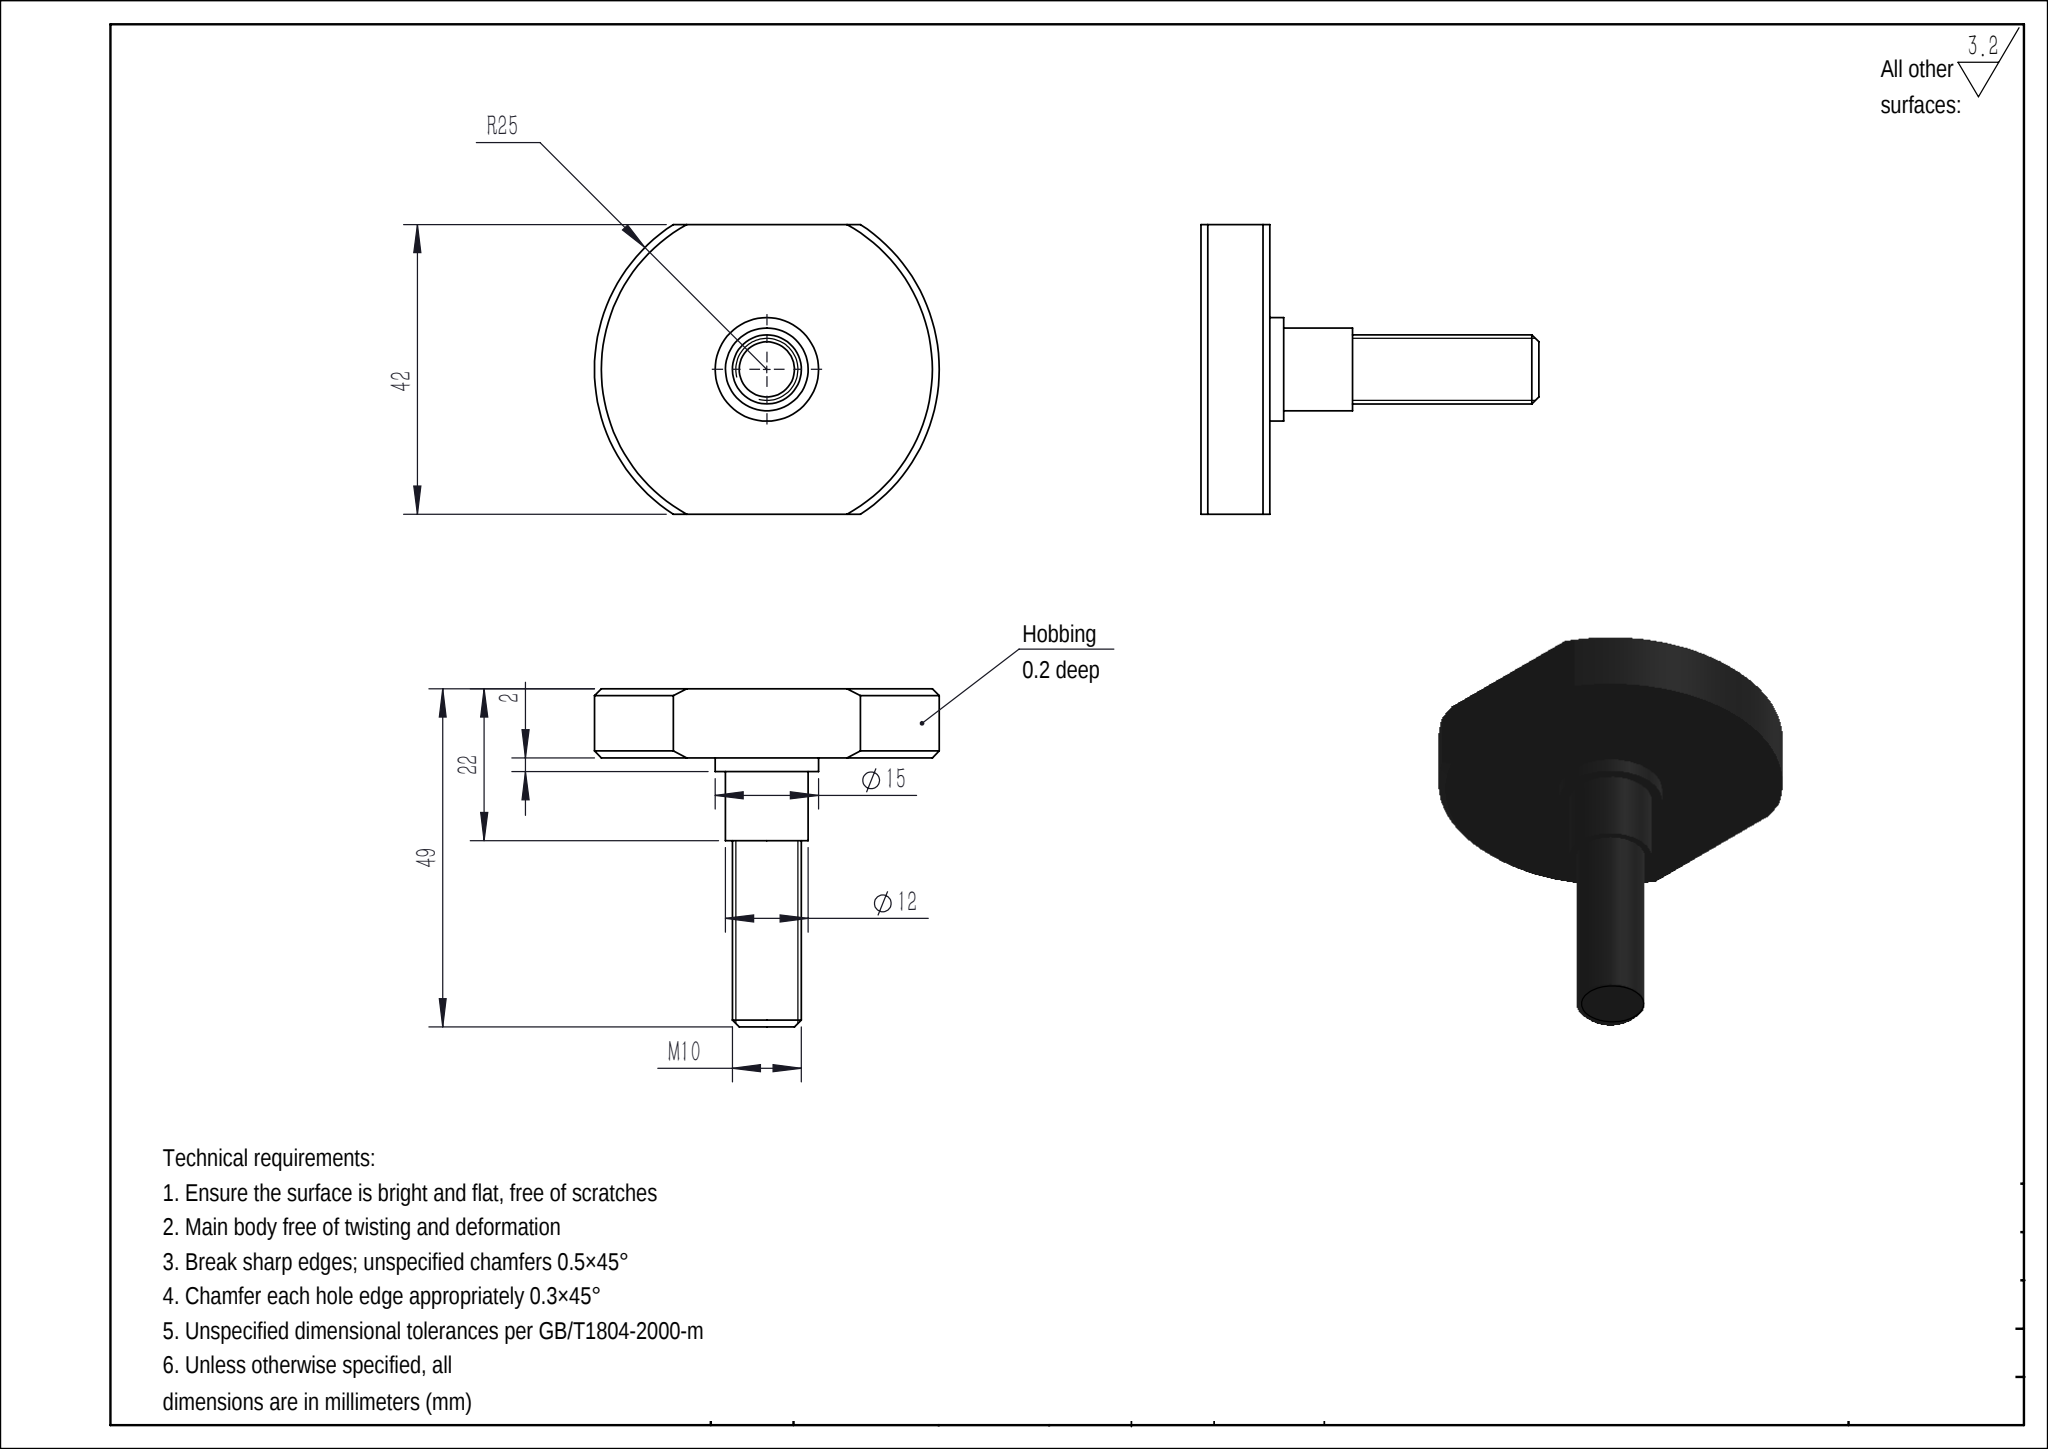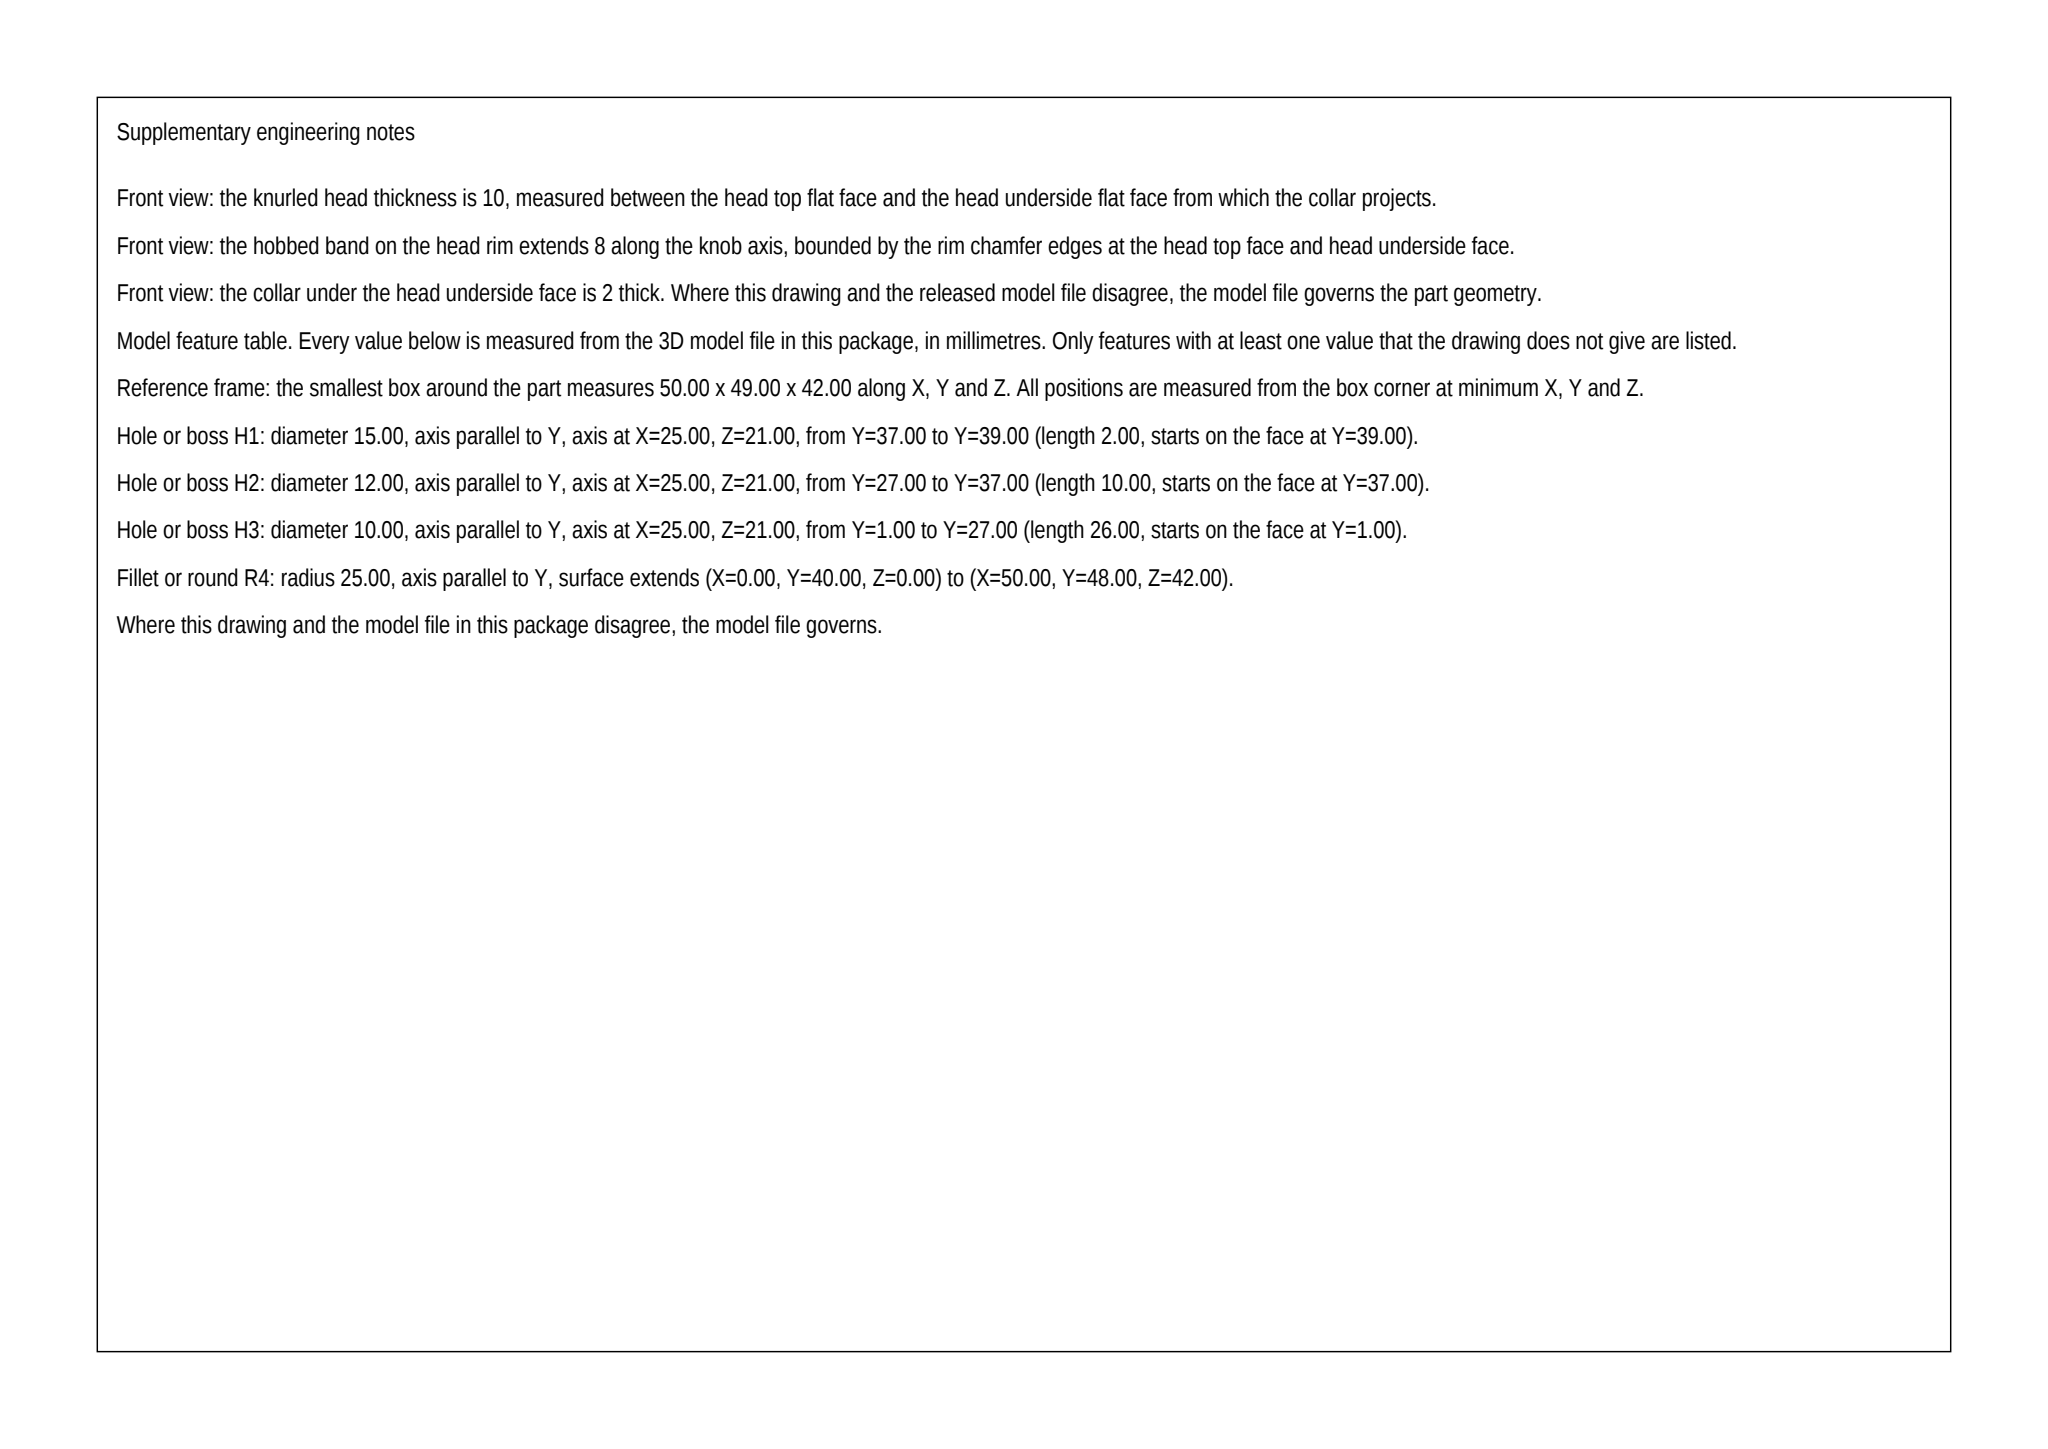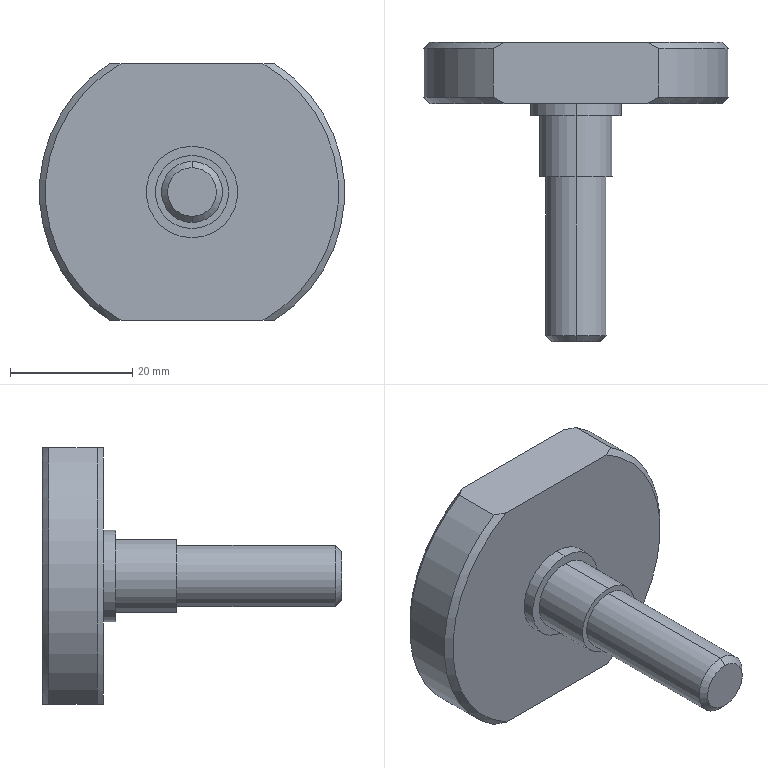Part | SolidWorks | mm | 1 solid | 21 faces | box 50 x 49 x 42 mm | volume 21653 mm3 | cylinder 8 | plane 7 | cone 6 | commonest cylinder face diameters 15 x2 12 x2 10 x2 50 x2
build123d program:
from build123d import *

# Parameters (mm, degrees)
SKETCH1_R           = 5
BOSS_EXTRUDE1_DEPTH = 27
SKETCH2_R           = 6
BOSS_EXTRUDE2_DEPTH = 12
SKETCH3_R           = 25
BOSS_EXTRUDE3_DEPTH = 10
CHAMFER1_SIZE       = 1
CHAMFER2_SIZE       = 1
SKETCH5_R           = 7.5
BOSS_EXTRUDE4_DEPTH = 2
SKETCH7_OUTSIDE_W   = 69.206
SKETCH7_OUTSIDE_H   = 69.206
SKETCH7_OUTSIDE_W_2 = 66.031
SKETCH7_OUTSIDE_H_2 = 42
CUT_EXTRUDE1_DEPTH  = 10


with BuildPart() as part:
    # Sketch1 → Boss-Extrude1 (new body)
    with BuildSketch(Plane(origin=(0, 0, 0), x_dir=(1, 0, 0), z_dir=(0, 1, 0))):
        with Locations(Location((0, 0, 0), (0, 0, 270))):
            Circle(SKETCH1_R)
    extrude(amount=BOSS_EXTRUDE1_DEPTH)

    # Sketch2 → Boss-Extrude2 (add)
    with BuildSketch(Plane(origin=(0, 27, 0), x_dir=(1, 0, 0), z_dir=(0, 1, 0))):
        with Locations(Location((0, 0, 0), (0, 0, 270))):
            Circle(SKETCH2_R)
    extrude(amount=BOSS_EXTRUDE2_DEPTH)

    # Sketch3 → Boss-Extrude3 (add)
    with BuildSketch(Plane(origin=(0, 39, 0), x_dir=(1, 0, 0), z_dir=(0, 1, 0))):
        with Locations(Location((0, 0, 0), (0, 0, 270))):
            Circle(SKETCH3_R)
    extrude(amount=BOSS_EXTRUDE3_DEPTH)

    # Chamfer1
    chamfer1_edges = [part.edges().sort_by_distance(p)[0] for p in [
        (0, 0, -5),
    ]]
    chamfer(chamfer1_edges, length=CHAMFER1_SIZE)

    # Chamfer2
    chamfer2_edges = [part.edges().sort_by_distance(p)[0] for p in [
        (0, 49, -25),
        (0, 39, -25),
    ]]
    chamfer(chamfer2_edges, length=CHAMFER2_SIZE)

    # Sketch5 → Boss-Extrude4 (add)
    with BuildSketch(Plane.XZ.offset(-39)):
        with Locations(Location((0, 0, 0), (0, 0, 90))):
            Circle(SKETCH5_R)
    extrude(amount=BOSS_EXTRUDE4_DEPTH)

    # Sketch7 outside → Cut-Extrude1 (cut)
    with BuildSketch(Plane(origin=(0, 49, 0), x_dir=(1, 0, 0), z_dir=(0, 1, 0))):
        Rectangle(SKETCH7_OUTSIDE_W, SKETCH7_OUTSIDE_H)
        Rectangle(SKETCH7_OUTSIDE_W_2, SKETCH7_OUTSIDE_H_2, mode=Mode.SUBTRACT)
    extrude(amount=-CUT_EXTRUDE1_DEPTH, mode=Mode.SUBTRACT)


solid = part.part
STEP:
#1=CARTESIAN_POINT('',(0.,37.,-7.5));
#2=VERTEX_POINT('',#1);
#3=CARTESIAN_POINT('',(0.,37.,7.5));
#4=VERTEX_POINT('',#3);
#5=CARTESIAN_POINT('',(0.,37.,0.));
#6=DIRECTION('',(0.,-1.,0.));
#7=DIRECTION('',(0.,0.,-1.));
#8=AXIS2_PLACEMENT_3D('',#5,#6,#7);
#9=CIRCLE('',#8,7.5);
#10=EDGE_CURVE('',#2,#4,#9,.T.);
#11=ORIENTED_EDGE('',*,*,#10,.F.);
#12=CARTESIAN_POINT('',(0.,39.,-7.5));
#13=VERTEX_POINT('',#12);
#14=CARTESIAN_POINT('',(0.,37.,-7.5));
#15=DIRECTION('',(0.,1.,0.));
#16=VECTOR('',#15,1000.);
#17=LINE('',#14,#16);
#18=EDGE_CURVE('',#2,#13,#17,.T.);
#19=ORIENTED_EDGE('',*,*,#18,.T.);
#20=CARTESIAN_POINT('',(0.,39.,7.5));
#21=VERTEX_POINT('',#20);
#22=CARTESIAN_POINT('',(0.,39.,0.));
#23=DIRECTION('',(0.,-1.,0.));
#24=DIRECTION('',(0.,0.,1.));
#25=AXIS2_PLACEMENT_3D('',#22,#23,#24);
#26=CIRCLE('',#25,7.5);
#27=EDGE_CURVE('',#13,#21,#26,.T.);
#28=ORIENTED_EDGE('',*,*,#27,.T.);
#29=CARTESIAN_POINT('',(0.,37.,7.5));
#30=DIRECTION('',(0.,1.,0.));
#31=VECTOR('',#30,1000.);
#32=LINE('',#29,#31);
#33=EDGE_CURVE('',#4,#21,#32,.T.);
#34=ORIENTED_EDGE('',*,*,#33,.F.);
#35=EDGE_LOOP('',(#11,#19,#28,#34));
#36=FACE_OUTER_BOUND('',#35,.T.);
#37=CARTESIAN_POINT('',(0.,37.,0.));
#38=DIRECTION('',(0.,1.,0.));
#39=DIRECTION('',(0.,0.,1.));
#40=AXIS2_PLACEMENT_3D('',#37,#38,#39);
#41=CYLINDRICAL_SURFACE('',#40,7.5);
#42=ADVANCED_FACE('',(#36),#41,.T.);
#43=CARTESIAN_POINT('',(0.,0.,-4.));
#44=VERTEX_POINT('',#43);
#45=CARTESIAN_POINT('',(0.,0.,4.));
#46=VERTEX_POINT('',#45);
#47=CARTESIAN_POINT('',(0.,0.,0.));
#48=DIRECTION('',(0.,-1.,0.));
#49=DIRECTION('',(0.,0.,1.));
#50=AXIS2_PLACEMENT_3D('',#47,#48,#49);
#51=CIRCLE('',#50,4.);
#52=EDGE_CURVE('',#44,#46,#51,.T.);
#53=ORIENTED_EDGE('',*,*,#52,.F.);
#54=CARTESIAN_POINT('',(0.,1.,-5.));
#55=VERTEX_POINT('',#54);
#56=CARTESIAN_POINT('',(0.,1.,-5.));
#57=DIRECTION('',(0.,0.7071,-0.7071));
#58=VECTOR('',#57,1000.);
#59=LINE('',#56,#58);
#60=EDGE_CURVE('',#44,#55,#59,.T.);
#61=ORIENTED_EDGE('',*,*,#60,.T.);
#62=CARTESIAN_POINT('',(0.,1.,5.));
#63=VERTEX_POINT('',#62);
#64=CARTESIAN_POINT('',(0.,1.,0.));
#65=DIRECTION('',(0.,1.,0.));
#66=DIRECTION('',(0.,0.,1.));
#67=AXIS2_PLACEMENT_3D('',#64,#65,#66);
#68=CIRCLE('',#67,5.);
#69=EDGE_CURVE('',#63,#55,#68,.T.);
#70=ORIENTED_EDGE('',*,*,#69,.F.);
#71=CARTESIAN_POINT('',(0.,1.,5.));
#72=DIRECTION('',(0.,0.7071,0.7071));
#73=VECTOR('',#72,1000.);
#74=LINE('',#71,#73);
#75=EDGE_CURVE('',#46,#63,#74,.T.);
#76=ORIENTED_EDGE('',*,*,#75,.F.);
#77=EDGE_LOOP('',(#53,#61,#70,#76));
#78=FACE_OUTER_BOUND('',#77,.T.);
#79=CARTESIAN_POINT('',(0.,1.,0.));
#80=DIRECTION('',(0.,1.,0.));
#81=DIRECTION('',(0.,0.,1.));
#82=AXIS2_PLACEMENT_3D('',#79,#80,#81);
#83=CONICAL_SURFACE('',#82,5.,0.7854);
#84=ADVANCED_FACE('',(#78),#83,.T.);
#85=CARTESIAN_POINT('',(0.,37.,-6.));
#86=VERTEX_POINT('',#85);
#87=CARTESIAN_POINT('',(0.,37.,6.));
#88=VERTEX_POINT('',#87);
#89=CARTESIAN_POINT('',(0.,37.,0.));
#90=DIRECTION('',(0.,-1.,0.));
#91=DIRECTION('',(0.,0.,-1.));
#92=AXIS2_PLACEMENT_3D('',#89,#90,#91);
#93=CIRCLE('',#92,6.);
#94=EDGE_CURVE('',#86,#88,#93,.T.);
#95=ORIENTED_EDGE('',*,*,#94,.T.);
#96=CARTESIAN_POINT('',(0.,27.,6.));
#97=VERTEX_POINT('',#96);
#98=CARTESIAN_POINT('',(0.,39.,6.));
#99=DIRECTION('',(0.,-1.,0.));
#100=VECTOR('',#99,1000.);
#101=LINE('',#98,#100);
#102=EDGE_CURVE('',#88,#97,#101,.T.);
#103=ORIENTED_EDGE('',*,*,#102,.T.);
#104=CARTESIAN_POINT('',(0.,27.,-6.));
#105=VERTEX_POINT('',#104);
#106=CARTESIAN_POINT('',(0.,27.,0.));
#107=DIRECTION('',(0.,1.,0.));
#108=DIRECTION('',(0.,0.,1.));
#109=AXIS2_PLACEMENT_3D('',#106,#107,#108);
#110=CIRCLE('',#109,6.);
#111=EDGE_CURVE('',#97,#105,#110,.T.);
#112=ORIENTED_EDGE('',*,*,#111,.T.);
#113=CARTESIAN_POINT('',(0.,39.,-6.));
#114=DIRECTION('',(0.,-1.,0.));
#115=VECTOR('',#114,1000.);
#116=LINE('',#113,#115);
#117=EDGE_CURVE('',#86,#105,#116,.T.);
#118=ORIENTED_EDGE('',*,*,#117,.F.);
#119=EDGE_LOOP('',(#95,#103,#112,#118));
#120=FACE_OUTER_BOUND('',#119,.T.);
#121=CARTESIAN_POINT('',(0.,39.,0.));
#122=DIRECTION('',(0.,-1.,0.));
#123=DIRECTION('',(0.,0.,-1.));
#124=AXIS2_PLACEMENT_3D('',#121,#122,#123);
#125=CYLINDRICAL_SURFACE('',#124,6.);
#126=ADVANCED_FACE('',(#120),#125,.T.);
#127=CARTESIAN_POINT('',(0.,27.,5.));
#128=VERTEX_POINT('',#127);
#129=CARTESIAN_POINT('',(0.,27.,-5.));
#130=VERTEX_POINT('',#129);
#131=CARTESIAN_POINT('',(0.,27.,0.));
#132=DIRECTION('',(0.,1.,0.));
#133=DIRECTION('',(0.,0.,1.));
#134=AXIS2_PLACEMENT_3D('',#131,#132,#133);
#135=CIRCLE('',#134,5.);
#136=EDGE_CURVE('',#128,#130,#135,.T.);
#137=ORIENTED_EDGE('',*,*,#136,.F.);
#138=CARTESIAN_POINT('',(0.,27.,5.));
#139=DIRECTION('',(0.,-1.,0.));
#140=VECTOR('',#139,1000.);
#141=LINE('',#138,#140);
#142=EDGE_CURVE('',#128,#63,#141,.T.);
#143=ORIENTED_EDGE('',*,*,#142,.T.);
#144=ORIENTED_EDGE('',*,*,#69,.T.);
#145=CARTESIAN_POINT('',(0.,27.,-5.));
#146=DIRECTION('',(0.,-1.,0.));
#147=VECTOR('',#146,1000.);
#148=LINE('',#145,#147);
#149=EDGE_CURVE('',#130,#55,#148,.T.);
#150=ORIENTED_EDGE('',*,*,#149,.F.);
#151=EDGE_LOOP('',(#137,#143,#144,#150));
#152=FACE_OUTER_BOUND('',#151,.T.);
#153=CARTESIAN_POINT('',(0.,27.,0.));
#154=DIRECTION('',(0.,-1.,0.));
#155=DIRECTION('',(0.,0.,-1.));
#156=AXIS2_PLACEMENT_3D('',#153,#154,#155);
#157=CYLINDRICAL_SURFACE('',#156,5.);
#158=ADVANCED_FACE('',(#152),#157,.T.);
#159=CARTESIAN_POINT('',(-11.619,49.,-21.));
#160=VERTEX_POINT('',#159);
#161=CARTESIAN_POINT('',(-11.619,49.,21.));
#162=VERTEX_POINT('',#161);
#163=CARTESIAN_POINT('',(0.,49.,0.));
#164=DIRECTION('',(0.,1.,0.));
#165=DIRECTION('',(0.,0.,1.));
#166=AXIS2_PLACEMENT_3D('',#163,#164,#165);
#167=CIRCLE('',#166,24.);
#168=EDGE_CURVE('',#160,#162,#167,.T.);
#169=ORIENTED_EDGE('',*,*,#168,.T.);
#170=CARTESIAN_POINT('',(11.619,49.,21.));
#171=VERTEX_POINT('',#170);
#172=CARTESIAN_POINT('',(-33.015,49.,21.));
#173=DIRECTION('',(1.,0.,0.));
#174=VECTOR('',#173,1000.);
#175=LINE('',#172,#174);
#176=EDGE_CURVE('',#162,#171,#175,.T.);
#177=ORIENTED_EDGE('',*,*,#176,.T.);
#178=CARTESIAN_POINT('',(11.619,49.,-21.));
#179=VERTEX_POINT('',#178);
#180=CARTESIAN_POINT('',(0.,49.,0.));
#181=DIRECTION('',(0.,1.,0.));
#182=DIRECTION('',(0.,0.,1.));
#183=AXIS2_PLACEMENT_3D('',#180,#181,#182);
#184=CIRCLE('',#183,24.);
#185=EDGE_CURVE('',#171,#179,#184,.T.);
#186=ORIENTED_EDGE('',*,*,#185,.T.);
#187=CARTESIAN_POINT('',(-33.015,49.,-21.));
#188=DIRECTION('',(-1.,0.,0.));
#189=VECTOR('',#188,1000.);
#190=LINE('',#187,#189);
#191=EDGE_CURVE('',#179,#160,#190,.T.);
#192=ORIENTED_EDGE('',*,*,#191,.T.);
#193=EDGE_LOOP('',(#169,#177,#186,#192));
#194=FACE_OUTER_BOUND('',#193,.T.);
#195=CARTESIAN_POINT('',(0.,49.,0.));
#196=DIRECTION('',(0.,1.,0.));
#197=DIRECTION('',(0.,0.,1.));
#198=AXIS2_PLACEMENT_3D('',#195,#196,#197);
#199=PLANE('',#198);
#200=ADVANCED_FACE('',(#194),#199,.T.);
#201=CARTESIAN_POINT('',(-13.565,48.,21.));
#202=VERTEX_POINT('',#201);
#203=CARTESIAN_POINT('',(-13.565,48.,-21.));
#204=VERTEX_POINT('',#203);
#205=CARTESIAN_POINT('',(0.,48.,0.));
#206=DIRECTION('',(0.,-1.,0.));
#207=DIRECTION('',(0.,0.,1.));
#208=AXIS2_PLACEMENT_3D('',#205,#206,#207);
#209=CIRCLE('',#208,25.);
#210=EDGE_CURVE('',#202,#204,#209,.T.);
#211=ORIENTED_EDGE('',*,*,#210,.F.);
#212=CARTESIAN_POINT('',(-13.565,48.,21.));
#213=CARTESIAN_POINT('',(-12.923,48.348,21.));
#214=CARTESIAN_POINT('',(-12.275,48.682,21.));
#215=CARTESIAN_POINT('',(-11.619,49.,21.));
#216=B_SPLINE_CURVE_WITH_KNOTS('',3,(#212,#213,#214,#215),.UNSPECIFIED.,.F.,.F.,(4,4),(0.04795,0.05014),.UNSPECIFIED.);
#217=EDGE_CURVE('',#202,#162,#216,.T.);
#218=ORIENTED_EDGE('',*,*,#217,.T.);
#219=ORIENTED_EDGE('',*,*,#168,.F.);
#220=CARTESIAN_POINT('',(-11.619,49.,-21.));
#221=CARTESIAN_POINT('',(-12.276,48.682,-21.));
#222=CARTESIAN_POINT('',(-12.924,48.347,-21.));
#223=CARTESIAN_POINT('',(-13.565,48.,-21.));
#224=B_SPLINE_CURVE_WITH_KNOTS('',3,(#220,#221,#222,#223),.UNSPECIFIED.,.F.,.F.,(4,4),(0.07437,0.07658),.UNSPECIFIED.);
#225=EDGE_CURVE('',#160,#204,#224,.T.);
#226=ORIENTED_EDGE('',*,*,#225,.T.);
#227=EDGE_LOOP('',(#211,#218,#219,#226));
#228=FACE_OUTER_BOUND('',#227,.T.);
#229=CARTESIAN_POINT('',(0.,49.,0.));
#230=DIRECTION('',(0.,-1.,0.));
#231=DIRECTION('',(0.,0.,-1.));
#232=AXIS2_PLACEMENT_3D('',#229,#230,#231);
#233=CONICAL_SURFACE('',#232,24.,0.7854);
#234=ADVANCED_FACE('',(#228),#233,.T.);
#235=ORIENTED_EDGE('',*,*,#185,.F.);
#236=CARTESIAN_POINT('',(13.565,48.,21.));
#237=VERTEX_POINT('',#236);
#238=CARTESIAN_POINT('',(11.619,49.,21.));
#239=CARTESIAN_POINT('',(12.276,48.682,21.));
#240=CARTESIAN_POINT('',(12.924,48.347,21.));
#241=CARTESIAN_POINT('',(13.565,48.,21.));
#242=B_SPLINE_CURVE_WITH_KNOTS('',3,(#238,#239,#240,#241),.UNSPECIFIED.,.F.,.F.,(4,4),(0.07437,0.07658),.UNSPECIFIED.);
#243=EDGE_CURVE('',#171,#237,#242,.T.);
#244=ORIENTED_EDGE('',*,*,#243,.T.);
#245=CARTESIAN_POINT('',(13.565,48.,-21.));
#246=VERTEX_POINT('',#245);
#247=CARTESIAN_POINT('',(0.,48.,0.));
#248=DIRECTION('',(0.,-1.,0.));
#249=DIRECTION('',(0.,0.,1.));
#250=AXIS2_PLACEMENT_3D('',#247,#248,#249);
#251=CIRCLE('',#250,25.);
#252=EDGE_CURVE('',#246,#237,#251,.T.);
#253=ORIENTED_EDGE('',*,*,#252,.F.);
#254=CARTESIAN_POINT('',(13.565,48.,-21.));
#255=CARTESIAN_POINT('',(12.923,48.348,-21.));
#256=CARTESIAN_POINT('',(12.275,48.682,-21.));
#257=CARTESIAN_POINT('',(11.619,49.,-21.));
#258=B_SPLINE_CURVE_WITH_KNOTS('',3,(#254,#255,#256,#257),.UNSPECIFIED.,.F.,.F.,(4,4),(0.04795,0.05014),.UNSPECIFIED.);
#259=EDGE_CURVE('',#246,#179,#258,.T.);
#260=ORIENTED_EDGE('',*,*,#259,.T.);
#261=EDGE_LOOP('',(#235,#244,#253,#260));
#262=FACE_OUTER_BOUND('',#261,.T.);
#263=CARTESIAN_POINT('',(0.,49.,0.));
#264=DIRECTION('',(0.,-1.,0.));
#265=DIRECTION('',(0.,0.,-1.));
#266=AXIS2_PLACEMENT_3D('',#263,#264,#265);
#267=CONICAL_SURFACE('',#266,24.,0.7854);
#268=ADVANCED_FACE('',(#262),#267,.T.);
#269=CARTESIAN_POINT('',(-13.565,40.,21.));
#270=VERTEX_POINT('',#269);
#271=CARTESIAN_POINT('',(-13.565,49.,21.));
#272=DIRECTION('',(0.,-1.,0.));
#273=VECTOR('',#272,1000.);
#274=LINE('',#271,#273);
#275=EDGE_CURVE('',#202,#270,#274,.T.);
#276=ORIENTED_EDGE('',*,*,#275,.F.);
#277=ORIENTED_EDGE('',*,*,#210,.T.);
#278=CARTESIAN_POINT('',(-13.565,40.,-21.));
#279=VERTEX_POINT('',#278);
#280=CARTESIAN_POINT('',(-13.565,49.,-21.));
#281=DIRECTION('',(0.,1.,0.));
#282=VECTOR('',#281,1000.);
#283=LINE('',#280,#282);
#284=EDGE_CURVE('',#279,#204,#283,.T.);
#285=ORIENTED_EDGE('',*,*,#284,.F.);
#286=CARTESIAN_POINT('',(0.,40.,0.));
#287=DIRECTION('',(0.,1.,0.));
#288=DIRECTION('',(0.,0.,1.));
#289=AXIS2_PLACEMENT_3D('',#286,#287,#288);
#290=CIRCLE('',#289,25.);
#291=EDGE_CURVE('',#279,#270,#290,.T.);
#292=ORIENTED_EDGE('',*,*,#291,.T.);
#293=EDGE_LOOP('',(#276,#277,#285,#292));
#294=FACE_OUTER_BOUND('',#293,.T.);
#295=CARTESIAN_POINT('',(0.,49.,0.));
#296=DIRECTION('',(0.,-1.,0.));
#297=DIRECTION('',(0.,0.,-1.));
#298=AXIS2_PLACEMENT_3D('',#295,#296,#297);
#299=CYLINDRICAL_SURFACE('',#298,25.);
#300=ADVANCED_FACE('',(#294),#299,.T.);
#301=CARTESIAN_POINT('',(13.565,40.,21.));
#302=VERTEX_POINT('',#301);
#303=CARTESIAN_POINT('',(13.565,49.,21.));
#304=DIRECTION('',(0.,1.,0.));
#305=VECTOR('',#304,1000.);
#306=LINE('',#303,#305);
#307=EDGE_CURVE('',#302,#237,#306,.T.);
#308=ORIENTED_EDGE('',*,*,#307,.F.);
#309=CARTESIAN_POINT('',(13.565,40.,-21.));
#310=VERTEX_POINT('',#309);
#311=CARTESIAN_POINT('',(0.,40.,0.));
#312=DIRECTION('',(0.,1.,0.));
#313=DIRECTION('',(0.,0.,1.));
#314=AXIS2_PLACEMENT_3D('',#311,#312,#313);
#315=CIRCLE('',#314,25.);
#316=EDGE_CURVE('',#302,#310,#315,.T.);
#317=ORIENTED_EDGE('',*,*,#316,.T.);
#318=CARTESIAN_POINT('',(13.565,49.,-21.));
#319=DIRECTION('',(0.,-1.,0.));
#320=VECTOR('',#319,1000.);
#321=LINE('',#318,#320);
#322=EDGE_CURVE('',#246,#310,#321,.T.);
#323=ORIENTED_EDGE('',*,*,#322,.F.);
#324=ORIENTED_EDGE('',*,*,#252,.T.);
#325=EDGE_LOOP('',(#308,#317,#323,#324));
#326=FACE_OUTER_BOUND('',#325,.T.);
#327=CARTESIAN_POINT('',(0.,49.,0.));
#328=DIRECTION('',(0.,-1.,0.));
#329=DIRECTION('',(0.,0.,-1.));
#330=AXIS2_PLACEMENT_3D('',#327,#328,#329);
#331=CYLINDRICAL_SURFACE('',#330,25.);
#332=ADVANCED_FACE('',(#326),#331,.T.);
#333=ORIENTED_EDGE('',*,*,#316,.F.);
#334=CARTESIAN_POINT('',(11.619,39.,21.));
#335=VERTEX_POINT('',#334);
#336=CARTESIAN_POINT('',(13.565,40.,21.));
#337=CARTESIAN_POINT('',(12.923,39.652,21.));
#338=CARTESIAN_POINT('',(12.275,39.318,21.));
#339=CARTESIAN_POINT('',(11.619,39.,21.));
#340=B_SPLINE_CURVE_WITH_KNOTS('',3,(#336,#337,#338,#339),.UNSPECIFIED.,.F.,.F.,(4,4),(0.04795,0.05014),.UNSPECIFIED.);
#341=EDGE_CURVE('',#302,#335,#340,.T.);
#342=ORIENTED_EDGE('',*,*,#341,.T.);
#343=CARTESIAN_POINT('',(11.619,39.,-21.));
#344=VERTEX_POINT('',#343);
#345=CARTESIAN_POINT('',(0.,39.,0.));
#346=DIRECTION('',(0.,-1.,0.));
#347=DIRECTION('',(0.,0.,1.));
#348=AXIS2_PLACEMENT_3D('',#345,#346,#347);
#349=CIRCLE('',#348,24.);
#350=EDGE_CURVE('',#344,#335,#349,.T.);
#351=ORIENTED_EDGE('',*,*,#350,.F.);
#352=CARTESIAN_POINT('',(11.619,39.,-21.));
#353=CARTESIAN_POINT('',(12.276,39.318,-21.));
#354=CARTESIAN_POINT('',(12.924,39.653,-21.));
#355=CARTESIAN_POINT('',(13.565,40.,-21.));
#356=B_SPLINE_CURVE_WITH_KNOTS('',3,(#352,#353,#354,#355),.UNSPECIFIED.,.F.,.F.,(4,4),(0.07437,0.07658),.UNSPECIFIED.);
#357=EDGE_CURVE('',#344,#310,#356,.T.);
#358=ORIENTED_EDGE('',*,*,#357,.T.);
#359=EDGE_LOOP('',(#333,#342,#351,#358));
#360=FACE_OUTER_BOUND('',#359,.T.);
#361=CARTESIAN_POINT('',(0.,40.,0.));
#362=DIRECTION('',(0.,1.,0.));
#363=DIRECTION('',(0.,0.,1.));
#364=AXIS2_PLACEMENT_3D('',#361,#362,#363);
#365=CONICAL_SURFACE('',#364,25.,0.7854);
#366=ADVANCED_FACE('',(#360),#365,.T.);
#367=CARTESIAN_POINT('',(-11.619,39.,21.));
#368=VERTEX_POINT('',#367);
#369=CARTESIAN_POINT('',(-11.619,39.,-21.));
#370=VERTEX_POINT('',#369);
#371=CARTESIAN_POINT('',(0.,39.,0.));
#372=DIRECTION('',(0.,-1.,0.));
#373=DIRECTION('',(0.,0.,1.));
#374=AXIS2_PLACEMENT_3D('',#371,#372,#373);
#375=CIRCLE('',#374,24.);
#376=EDGE_CURVE('',#368,#370,#375,.T.);
#377=ORIENTED_EDGE('',*,*,#376,.F.);
#378=CARTESIAN_POINT('',(-11.619,39.,21.));
#379=CARTESIAN_POINT('',(-12.276,39.318,21.));
#380=CARTESIAN_POINT('',(-12.924,39.653,21.));
#381=CARTESIAN_POINT('',(-13.565,40.,21.));
#382=B_SPLINE_CURVE_WITH_KNOTS('',3,(#378,#379,#380,#381),.UNSPECIFIED.,.F.,.F.,(4,4),(0.07437,0.07658),.UNSPECIFIED.);
#383=EDGE_CURVE('',#368,#270,#382,.T.);
#384=ORIENTED_EDGE('',*,*,#383,.T.);
#385=ORIENTED_EDGE('',*,*,#291,.F.);
#386=CARTESIAN_POINT('',(-13.565,40.,-21.));
#387=CARTESIAN_POINT('',(-12.923,39.652,-21.));
#388=CARTESIAN_POINT('',(-12.275,39.318,-21.));
#389=CARTESIAN_POINT('',(-11.619,39.,-21.));
#390=B_SPLINE_CURVE_WITH_KNOTS('',3,(#386,#387,#388,#389),.UNSPECIFIED.,.F.,.F.,(4,4),(0.04795,0.05014),.UNSPECIFIED.);
#391=EDGE_CURVE('',#279,#370,#390,.T.);
#392=ORIENTED_EDGE('',*,*,#391,.T.);
#393=EDGE_LOOP('',(#377,#384,#385,#392));
#394=FACE_OUTER_BOUND('',#393,.T.);
#395=CARTESIAN_POINT('',(0.,40.,0.));
#396=DIRECTION('',(0.,1.,0.));
#397=DIRECTION('',(0.,0.,1.));
#398=AXIS2_PLACEMENT_3D('',#395,#396,#397);
#399=CONICAL_SURFACE('',#398,25.,0.7854);
#400=ADVANCED_FACE('',(#394),#399,.T.);
#401=CARTESIAN_POINT('',(0.,39.,0.));
#402=DIRECTION('',(0.,-1.,0.));
#403=DIRECTION('',(0.,0.,1.));
#404=AXIS2_PLACEMENT_3D('',#401,#402,#403);
#405=CIRCLE('',#404,7.5);
#406=EDGE_CURVE('',#21,#13,#405,.T.);
#407=ORIENTED_EDGE('',*,*,#406,.F.);
#408=ORIENTED_EDGE('',*,*,#27,.F.);
#409=EDGE_LOOP('',(#407,#408));
#410=FACE_BOUND('',#409,.T.);
#411=CARTESIAN_POINT('',(0.,39.,21.));
#412=DIRECTION('',(1.,0.,0.));
#413=VECTOR('',#412,1000.);
#414=LINE('',#411,#413);
#415=EDGE_CURVE('',#368,#335,#414,.T.);
#416=ORIENTED_EDGE('',*,*,#415,.F.);
#417=ORIENTED_EDGE('',*,*,#376,.T.);
#418=CARTESIAN_POINT('',(0.,39.,-21.));
#419=DIRECTION('',(-1.,0.,0.));
#420=VECTOR('',#419,1000.);
#421=LINE('',#418,#420);
#422=EDGE_CURVE('',#344,#370,#421,.T.);
#423=ORIENTED_EDGE('',*,*,#422,.F.);
#424=ORIENTED_EDGE('',*,*,#350,.T.);
#425=EDGE_LOOP('',(#416,#417,#423,#424));
#426=FACE_OUTER_BOUND('',#425,.T.);
#427=CARTESIAN_POINT('',(0.,39.,0.));
#428=DIRECTION('',(0.,1.,0.));
#429=DIRECTION('',(0.,0.,1.));
#430=AXIS2_PLACEMENT_3D('',#427,#428,#429);
#431=PLANE('',#430);
#432=ADVANCED_FACE('',(#410,#426),#431,.F.);
#433=ORIENTED_EDGE('',*,*,#142,.F.);
#434=CARTESIAN_POINT('',(0.,27.,0.));
#435=DIRECTION('',(0.,1.,0.));
#436=DIRECTION('',(0.,0.,1.));
#437=AXIS2_PLACEMENT_3D('',#434,#435,#436);
#438=CIRCLE('',#437,5.);
#439=EDGE_CURVE('',#130,#128,#438,.T.);
#440=ORIENTED_EDGE('',*,*,#439,.F.);
#441=ORIENTED_EDGE('',*,*,#149,.T.);
#442=CARTESIAN_POINT('',(0.,1.,0.));
#443=DIRECTION('',(0.,1.,0.));
#444=DIRECTION('',(0.,0.,1.));
#445=AXIS2_PLACEMENT_3D('',#442,#443,#444);
#446=CIRCLE('',#445,5.);
#447=EDGE_CURVE('',#55,#63,#446,.T.);
#448=ORIENTED_EDGE('',*,*,#447,.T.);
#449=EDGE_LOOP('',(#433,#440,#441,#448));
#450=FACE_OUTER_BOUND('',#449,.T.);
#451=CARTESIAN_POINT('',(0.,27.,0.));
#452=DIRECTION('',(0.,-1.,0.));
#453=DIRECTION('',(0.,0.,-1.));
#454=AXIS2_PLACEMENT_3D('',#451,#452,#453);
#455=CYLINDRICAL_SURFACE('',#454,5.);
#456=ADVANCED_FACE('',(#450),#455,.T.);
#457=CARTESIAN_POINT('',(0.,0.,0.));
#458=DIRECTION('',(0.,-1.,0.));
#459=DIRECTION('',(0.,0.,1.));
#460=AXIS2_PLACEMENT_3D('',#457,#458,#459);
#461=CIRCLE('',#460,4.);
#462=EDGE_CURVE('',#46,#44,#461,.T.);
#463=ORIENTED_EDGE('',*,*,#462,.T.);
#464=ORIENTED_EDGE('',*,*,#52,.T.);
#465=EDGE_LOOP('',(#463,#464));
#466=FACE_OUTER_BOUND('',#465,.T.);
#467=CARTESIAN_POINT('',(0.,0.,0.));
#468=DIRECTION('',(0.,1.,0.));
#469=DIRECTION('',(0.,0.,1.));
#470=AXIS2_PLACEMENT_3D('',#467,#468,#469);
#471=PLANE('',#470);
#472=ADVANCED_FACE('',(#466),#471,.F.);
#473=CARTESIAN_POINT('',(0.,27.,0.));
#474=DIRECTION('',(0.,1.,0.));
#475=DIRECTION('',(0.,0.,1.));
#476=AXIS2_PLACEMENT_3D('',#473,#474,#475);
#477=CIRCLE('',#476,6.);
#478=EDGE_CURVE('',#105,#97,#477,.T.);
#479=ORIENTED_EDGE('',*,*,#478,.F.);
#480=ORIENTED_EDGE('',*,*,#111,.F.);
#481=EDGE_LOOP('',(#479,#480));
#482=FACE_OUTER_BOUND('',#481,.T.);
#483=ORIENTED_EDGE('',*,*,#439,.T.);
#484=ORIENTED_EDGE('',*,*,#136,.T.);
#485=EDGE_LOOP('',(#483,#484));
#486=FACE_BOUND('',#485,.T.);
#487=CARTESIAN_POINT('',(0.,27.,0.));
#488=DIRECTION('',(0.,1.,0.));
#489=DIRECTION('',(0.,0.,1.));
#490=AXIS2_PLACEMENT_3D('',#487,#488,#489);
#491=PLANE('',#490);
#492=ADVANCED_FACE('',(#482,#486),#491,.F.);
#493=ORIENTED_EDGE('',*,*,#102,.F.);
#494=CARTESIAN_POINT('',(0.,37.,0.));
#495=DIRECTION('',(0.,-1.,0.));
#496=DIRECTION('',(0.,0.,-1.));
#497=AXIS2_PLACEMENT_3D('',#494,#495,#496);
#498=CIRCLE('',#497,6.);
#499=EDGE_CURVE('',#88,#86,#498,.T.);
#500=ORIENTED_EDGE('',*,*,#499,.T.);
#501=ORIENTED_EDGE('',*,*,#117,.T.);
#502=ORIENTED_EDGE('',*,*,#478,.T.);
#503=EDGE_LOOP('',(#493,#500,#501,#502));
#504=FACE_OUTER_BOUND('',#503,.T.);
#505=CARTESIAN_POINT('',(0.,39.,0.));
#506=DIRECTION('',(0.,-1.,0.));
#507=DIRECTION('',(0.,0.,-1.));
#508=AXIS2_PLACEMENT_3D('',#505,#506,#507);
#509=CYLINDRICAL_SURFACE('',#508,6.);
#510=ADVANCED_FACE('',(#504),#509,.T.);
#511=ORIENTED_EDGE('',*,*,#60,.F.);
#512=ORIENTED_EDGE('',*,*,#462,.F.);
#513=ORIENTED_EDGE('',*,*,#75,.T.);
#514=ORIENTED_EDGE('',*,*,#447,.F.);
#515=EDGE_LOOP('',(#511,#512,#513,#514));
#516=FACE_OUTER_BOUND('',#515,.T.);
#517=CARTESIAN_POINT('',(0.,1.,0.));
#518=DIRECTION('',(0.,1.,0.));
#519=DIRECTION('',(0.,0.,1.));
#520=AXIS2_PLACEMENT_3D('',#517,#518,#519);
#521=CONICAL_SURFACE('',#520,5.,0.7854);
#522=ADVANCED_FACE('',(#516),#521,.T.);
#523=CARTESIAN_POINT('',(0.,37.,0.));
#524=DIRECTION('',(0.,-1.,0.));
#525=DIRECTION('',(0.,0.,-1.));
#526=AXIS2_PLACEMENT_3D('',#523,#524,#525);
#527=CIRCLE('',#526,7.5);
#528=EDGE_CURVE('',#4,#2,#527,.T.);
#529=ORIENTED_EDGE('',*,*,#528,.T.);
#530=ORIENTED_EDGE('',*,*,#10,.T.);
#531=EDGE_LOOP('',(#529,#530));
#532=FACE_OUTER_BOUND('',#531,.T.);
#533=ORIENTED_EDGE('',*,*,#94,.F.);
#534=ORIENTED_EDGE('',*,*,#499,.F.);
#535=EDGE_LOOP('',(#533,#534));
#536=FACE_BOUND('',#535,.T.);
#537=CARTESIAN_POINT('',(0.,37.,0.));
#538=DIRECTION('',(0.,-1.,0.));
#539=DIRECTION('',(0.,0.,-1.));
#540=AXIS2_PLACEMENT_3D('',#537,#538,#539);
#541=PLANE('',#540);
#542=ADVANCED_FACE('',(#532,#536),#541,.T.);
#543=ORIENTED_EDGE('',*,*,#18,.F.);
#544=ORIENTED_EDGE('',*,*,#528,.F.);
#545=ORIENTED_EDGE('',*,*,#33,.T.);
#546=ORIENTED_EDGE('',*,*,#406,.T.);
#547=EDGE_LOOP('',(#543,#544,#545,#546));
#548=FACE_OUTER_BOUND('',#547,.T.);
#549=CARTESIAN_POINT('',(0.,37.,0.));
#550=DIRECTION('',(0.,1.,0.));
#551=DIRECTION('',(0.,0.,1.));
#552=AXIS2_PLACEMENT_3D('',#549,#550,#551);
#553=CYLINDRICAL_SURFACE('',#552,7.5);
#554=ADVANCED_FACE('',(#548),#553,.T.);
#555=ORIENTED_EDGE('',*,*,#191,.F.);
#556=ORIENTED_EDGE('',*,*,#259,.F.);
#557=ORIENTED_EDGE('',*,*,#322,.T.);
#558=ORIENTED_EDGE('',*,*,#357,.F.);
#559=ORIENTED_EDGE('',*,*,#422,.T.);
#560=ORIENTED_EDGE('',*,*,#391,.F.);
#561=ORIENTED_EDGE('',*,*,#284,.T.);
#562=ORIENTED_EDGE('',*,*,#225,.F.);
#563=EDGE_LOOP('',(#555,#556,#557,#558,#559,#560,#561,#562));
#564=FACE_OUTER_BOUND('',#563,.T.);
#565=CARTESIAN_POINT('',(-33.015,39.,-21.));
#566=DIRECTION('',(0.,0.,-1.));
#567=DIRECTION('',(-1.,0.,0.));
#568=AXIS2_PLACEMENT_3D('',#565,#566,#567);
#569=PLANE('',#568);
#570=ADVANCED_FACE('',(#564),#569,.T.);
#571=ORIENTED_EDGE('',*,*,#176,.F.);
#572=ORIENTED_EDGE('',*,*,#217,.F.);
#573=ORIENTED_EDGE('',*,*,#275,.T.);
#574=ORIENTED_EDGE('',*,*,#383,.F.);
#575=ORIENTED_EDGE('',*,*,#415,.T.);
#576=ORIENTED_EDGE('',*,*,#341,.F.);
#577=ORIENTED_EDGE('',*,*,#307,.T.);
#578=ORIENTED_EDGE('',*,*,#243,.F.);
#579=EDGE_LOOP('',(#571,#572,#573,#574,#575,#576,#577,#578));
#580=FACE_OUTER_BOUND('',#579,.T.);
#581=CARTESIAN_POINT('',(-33.015,39.,21.));
#582=DIRECTION('',(0.,0.,1.));
#583=DIRECTION('',(1.,0.,0.));
#584=AXIS2_PLACEMENT_3D('',#581,#582,#583);
#585=PLANE('',#584);
#586=ADVANCED_FACE('',(#580),#585,.T.);
#587=CLOSED_SHELL('',(#42,#84,#126,#158,#200,#234,#268,#300,#332,#366,#400,#432,#456,#472,#492,#510,#522,#542,#554,#570,#586));
#588=MANIFOLD_SOLID_BREP('',#587);
#589=CARTESIAN_POINT('',(0.,0.,0.));
#590=DIRECTION('',(0.,0.,1.));
#591=DIRECTION('',(1.,0.,0.));
#592=AXIS2_PLACEMENT_3D('',#589,#590,#591);
#593=(LENGTH_UNIT()NAMED_UNIT(*)SI_UNIT(.MILLI.,.METRE.));
#594=UNCERTAINTY_MEASURE_WITH_UNIT(LENGTH_MEASURE(0.00001),#593,'','');
#595=(NAMED_UNIT(*)PLANE_ANGLE_UNIT()SI_UNIT($,.RADIAN.));
#596=(NAMED_UNIT(*)SI_UNIT($,.STERADIAN.)SOLID_ANGLE_UNIT());
#597=(GEOMETRIC_REPRESENTATION_CONTEXT(3)GLOBAL_UNCERTAINTY_ASSIGNED_CONTEXT((#594))GLOBAL_UNIT_ASSIGNED_CONTEXT((#593,#595,#596))REPRESENTATION_CONTEXT('',''));
#598=ADVANCED_BREP_SHAPE_REPRESENTATION('',(#588,#592),#597);